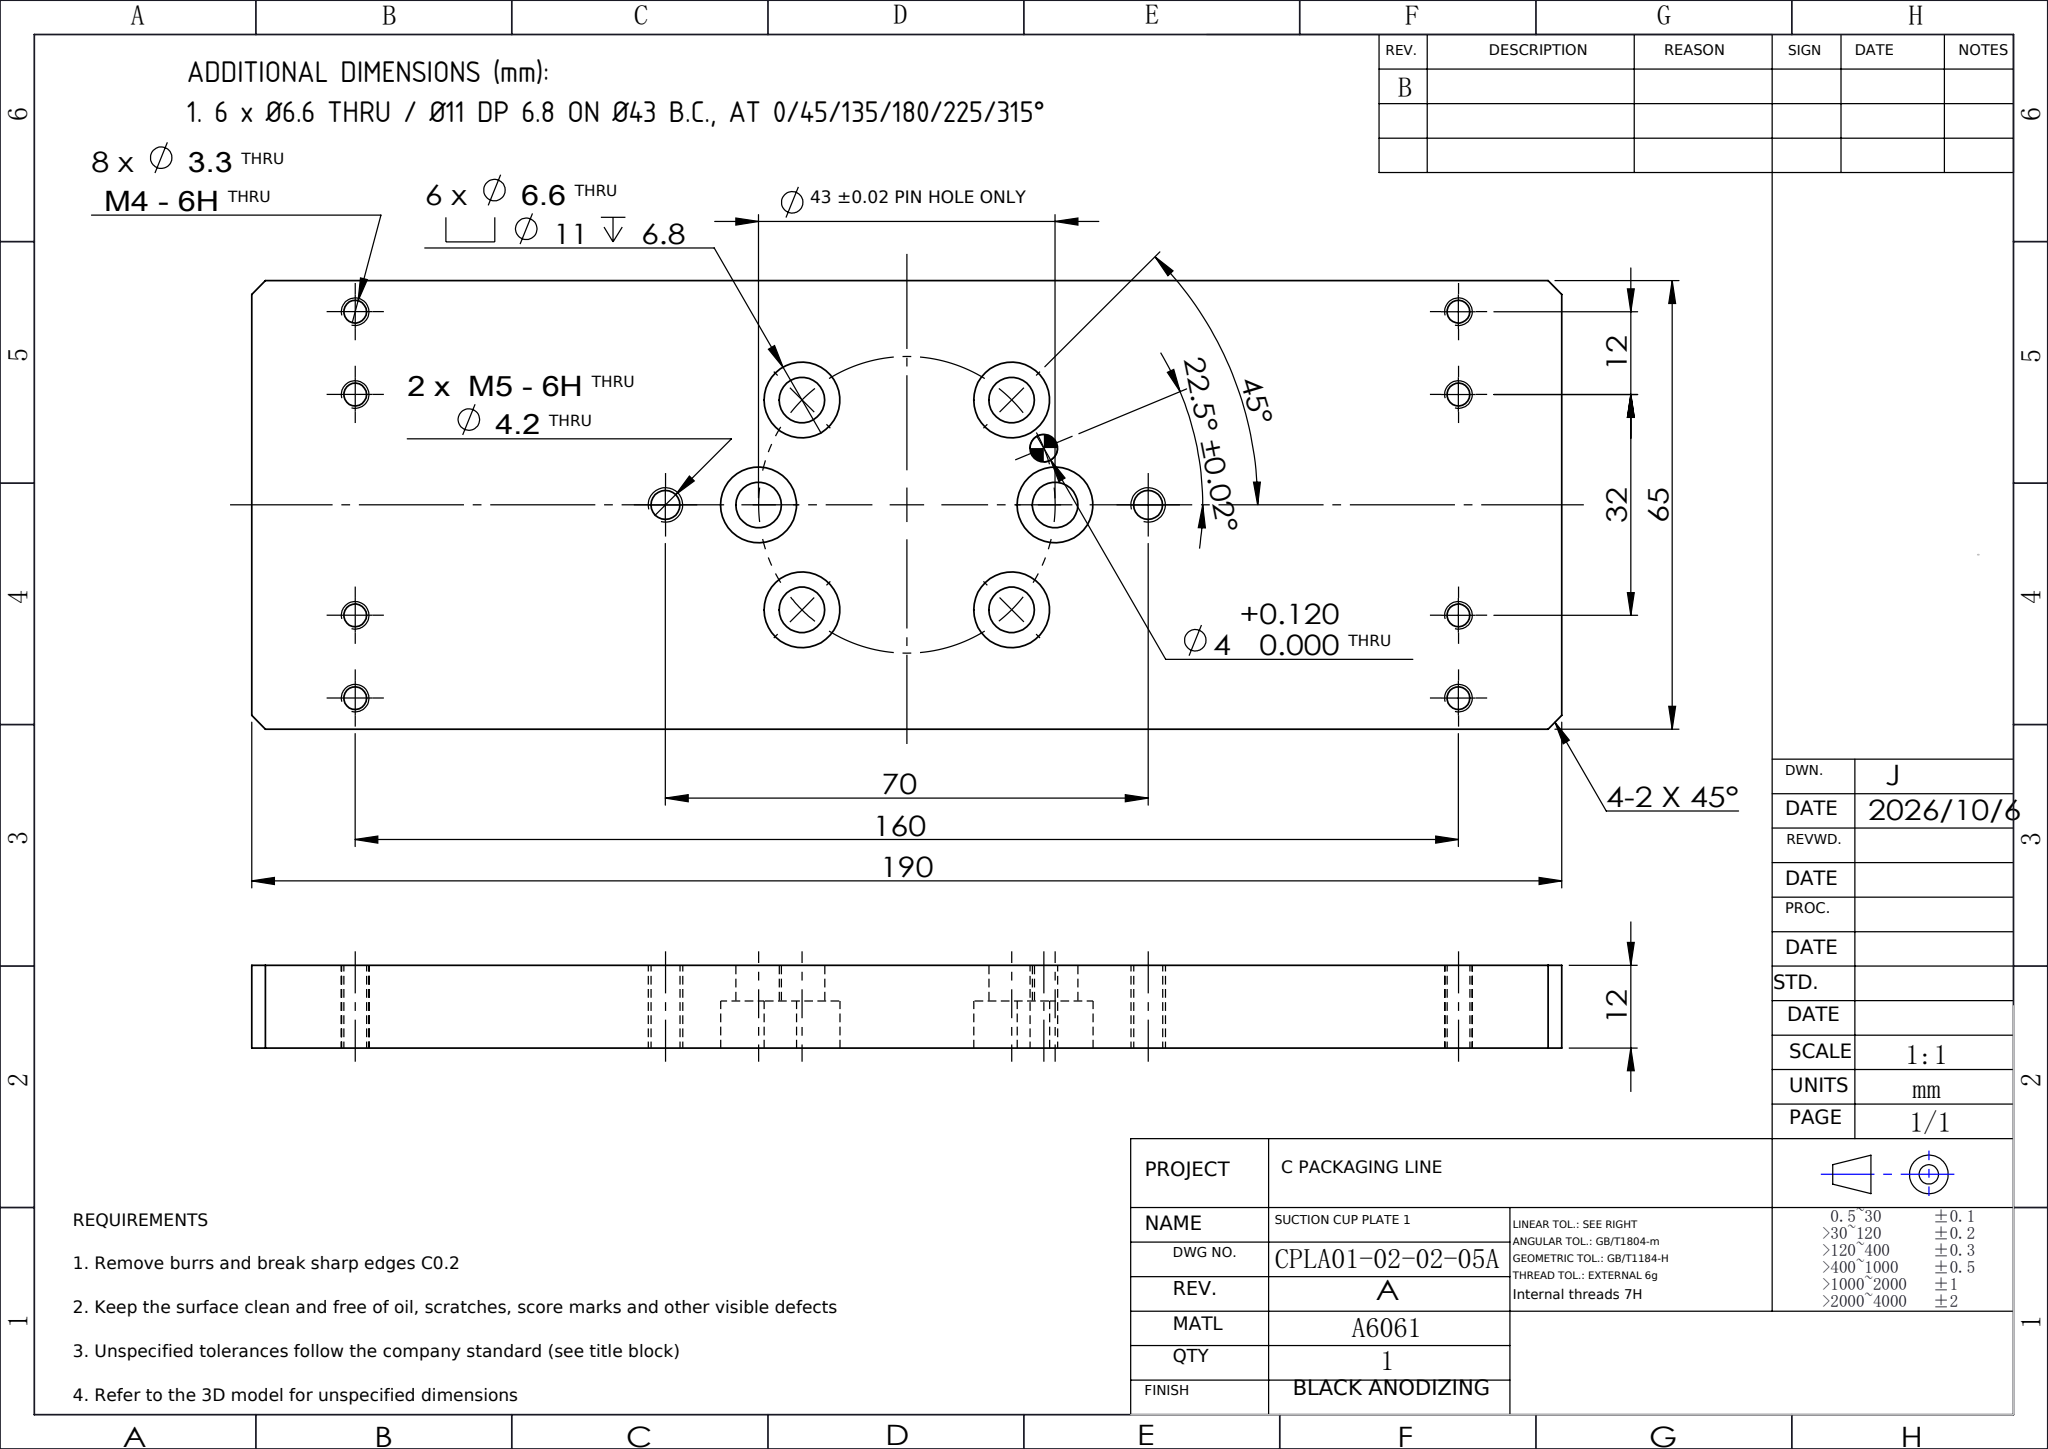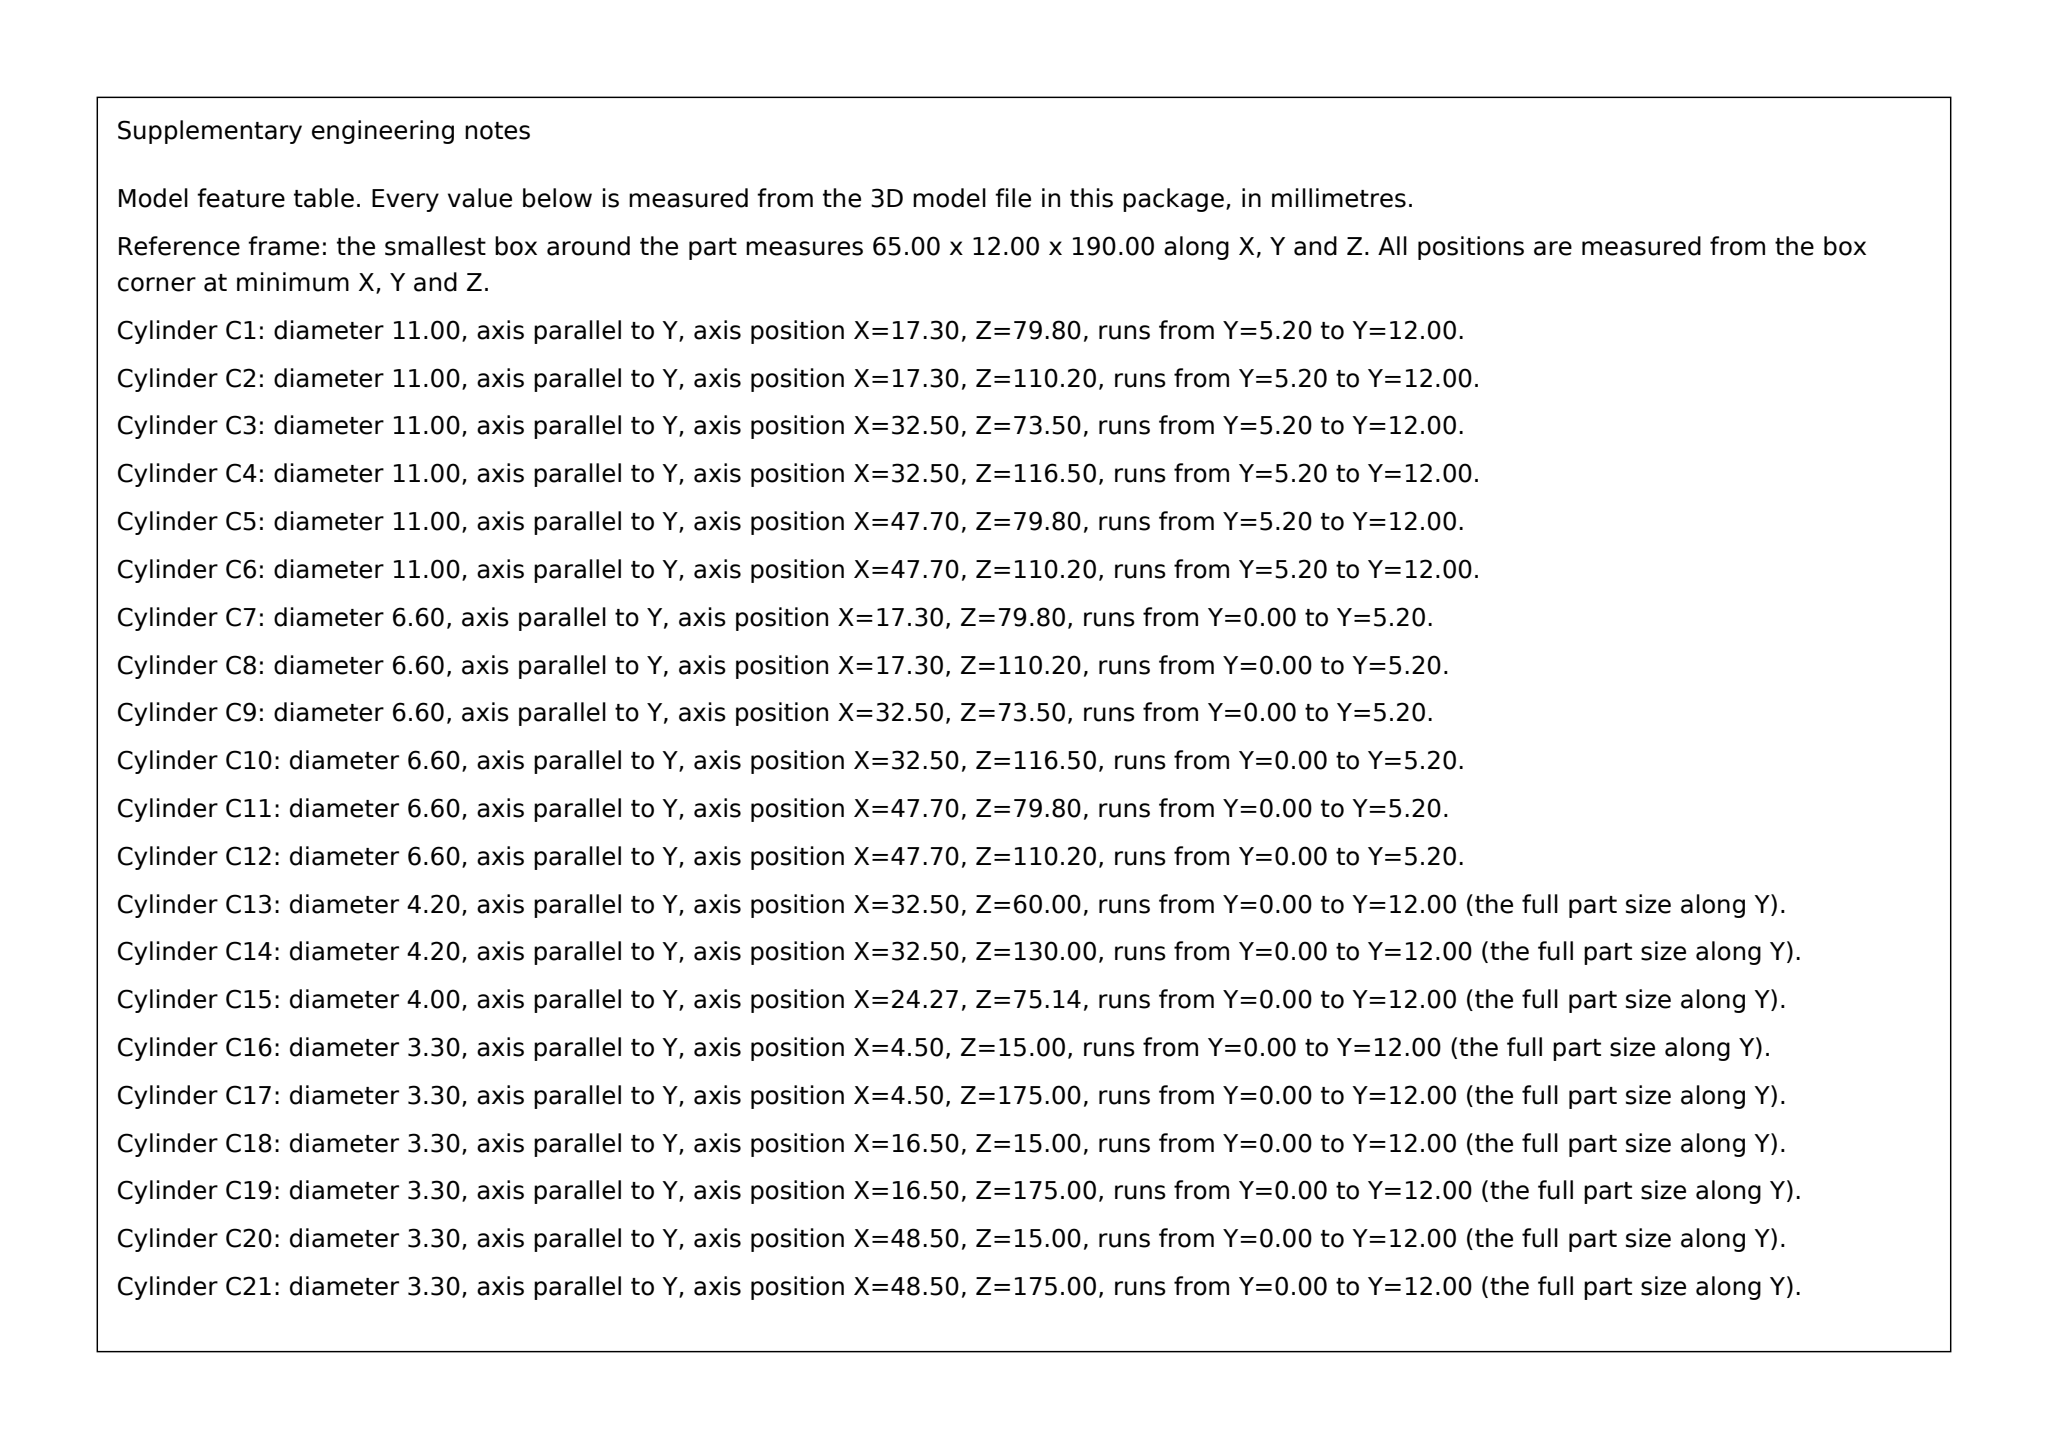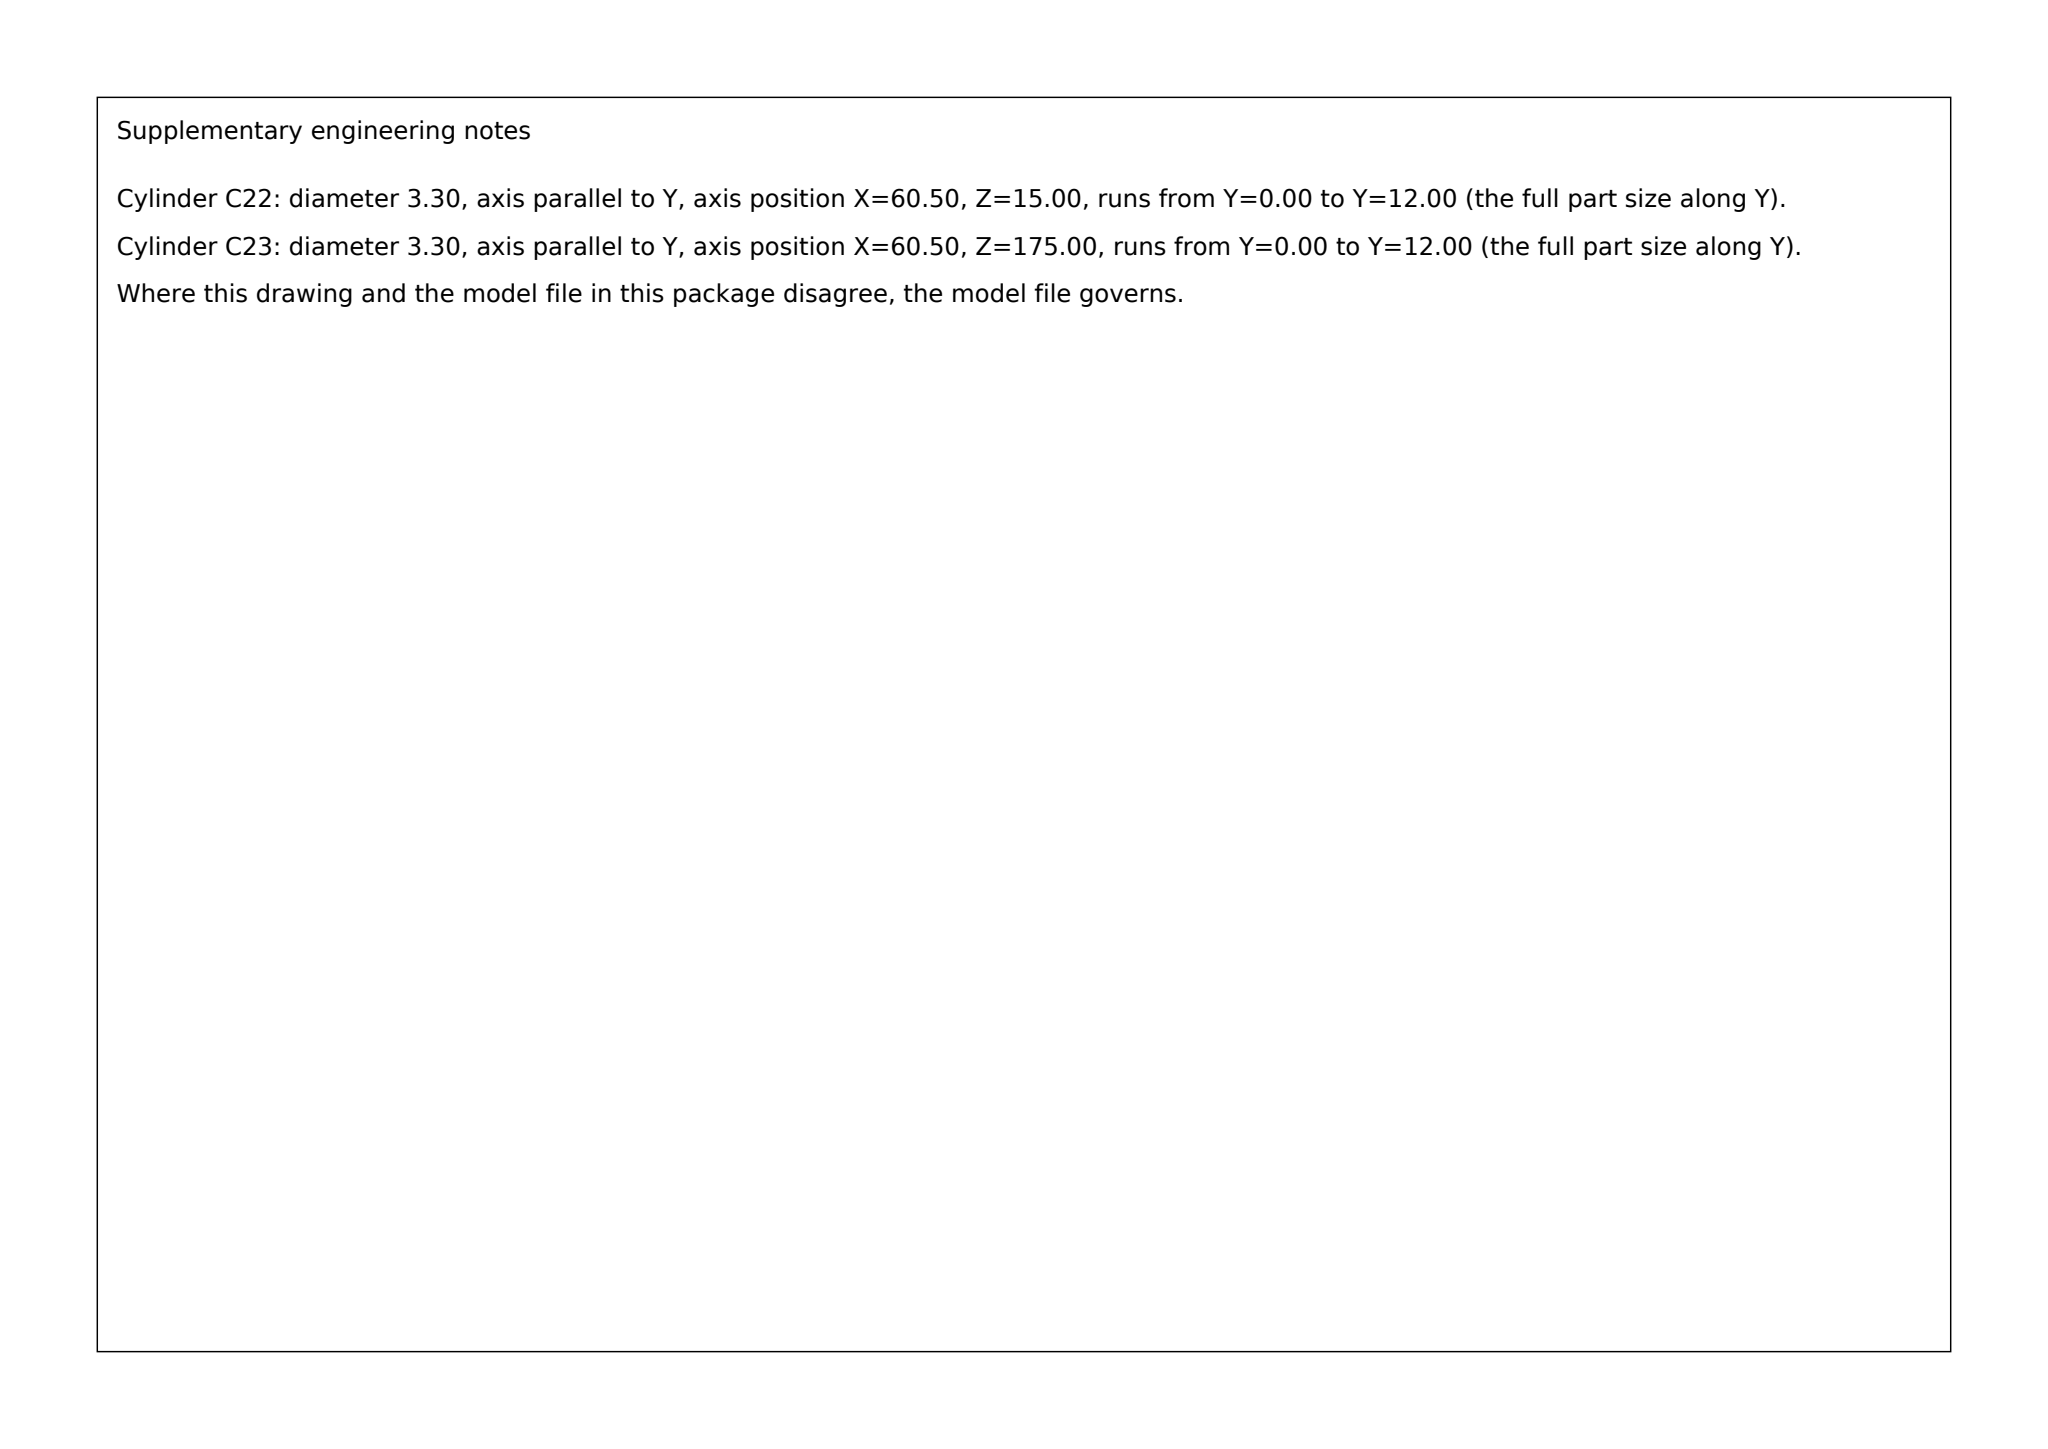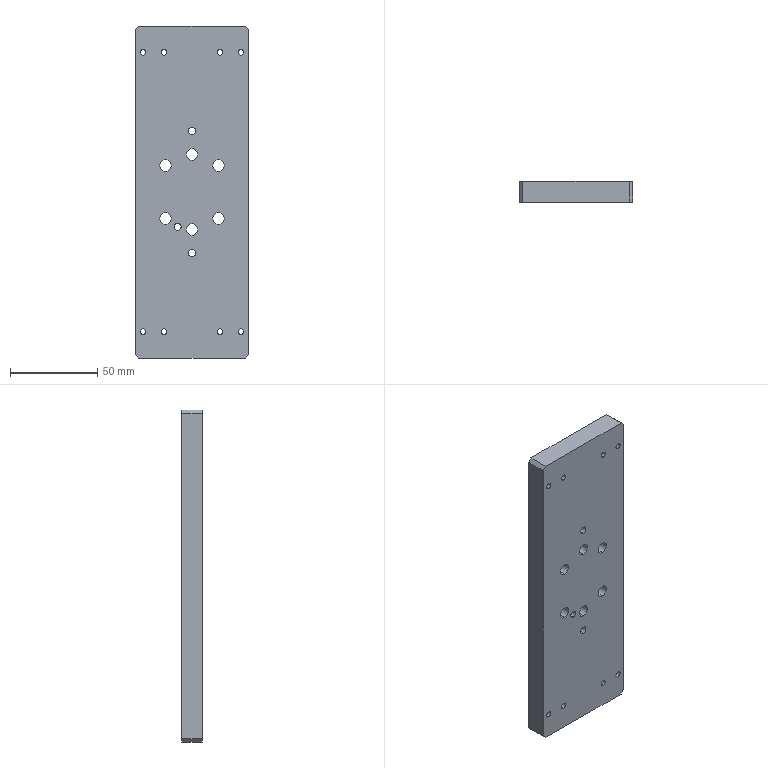Part | SolidWorks | mm | 1 solid | 62 faces | box 65 x 12 x 190 mm | volume 141855 mm3 | cylinder 46 | plane 16 | commonest cylinder face diameters 3.3 x16 11 x12 6.6 x12 4.2 x4 4 x2
build123d program:
from build123d import *

# Parameters (mm, degrees)
SKETCH1_W                                       = 120
SKETCH1_H                                       = 295
BOSS_EXTRUDE1_DEPTH                             = 12
SKETCH2_W                                       = 280
SKETCH2_H                                       = 12
BOSS_EXTRUDE2_DEPTH                             = 55
SKETCH3_R                                       = 6.5
CUT_EXTRUDE1_DEPTH                              = 188.417
LPATTERN1_COUNT                                 = 4
LPATTERN1_PITCH                                 = 68
SKETCH4_W                                       = 12
SKETCH4_H                                       = 2
CUT_EXTRUDE2_DEPTH                              = 230.184
M5_HEX_SOCKET_HEAD_CAP_SCREW_CBORE2_D           = 5.5
M5_HEX_SOCKET_HEAD_CAP_SCREW_CBORE2_CBORE_D     = 10
M5_HEX_SOCKET_HEAD_CAP_SCREW_CBORE2_CBORE_DEPTH = 5.4
SKETCH15_W                                      = 140
SKETCH15_H                                      = 354.743
SKETCH15_W_2                                    = 206.533
SKETCH15_H_2                                    = 375.74
CUT_EXTRUDE3_DEPTH                              = 188.417
SKETCH16_W                                      = 25
SKETCH16_H                                      = 520
CUT_EXTRUDE4_DEPTH                              = 155.678
CHAMFER1_SIZE                                   = 2
FILLET1_R                                       = 5
M4_TAPPED_HOLE1_D                               = 3.3
LPATTERN2_COUNT                                 = 2
LPATTERN2_PITCH                                 = 160
M4_TAPPED_HOLE2_D                               = 3.3
F_5_0MM_DOWEL_PIN_HOLE1_D                       = 5
SKETCH28_W                                      = 171.475
SKETCH28_H                                      = 89.112
CUT_EXTRUDE5_DEPTH                              = 155.678
CHAMFER2_SIZE                                   = 2
SKETCH29_W                                      = 120.267
SKETCH29_H                                      = 29.757
SKETCH29_W_2                                    = 113.82
SKETCH29_H_2                                    = 23.557
CUT_EXTRUDE6_DEPTH                              = 152.514
CHAMFER3_SIZE                                   = 2
SKETCH30_W                                      = 37.387
SKETCH30_H                                      = 12.641
SKETCH30_W_2                                    = 6.59
SKETCH30_H_2                                    = 8.943
SKETCH30_W_3                                    = 6.724
SKETCH30_H_3                                    = 9.279
BOSS_EXTRUDE3_DEPTH                             = 12
M6_HEX_SOCKET_HEAD_CAP_SCREW_CBORE1_D           = 6.6
M6_HEX_SOCKET_HEAD_CAP_SCREW_CBORE1_CBORE_D     = 11
M6_HEX_SOCKET_HEAD_CAP_SCREW_CBORE1_CBORE_DEPTH = 6.8
SKETCH33_R                                      = 2
CUT_EXTRUDE7_DEPTH                              = 133.123
M5_TAPPED_HOLE1_D                               = 4.2


with BuildPart() as part:
    # Sketch1 → Boss-Extrude1 (new body)
    with BuildSketch(Plane(origin=(0, 0, 0), x_dir=(1, 0, 0), z_dir=(0, 1, 0))):
        Rectangle(SKETCH1_W, SKETCH1_H)
    extrude(amount=BOSS_EXTRUDE1_DEPTH)

    # Sketch2 → Boss-Extrude2 (add)
    with BuildSketch(Plane(origin=(60, 0, 0), x_dir=(0, 0, -1), z_dir=(1, 0, 0))):
        with Locations((-7.5, 6)):
            Rectangle(SKETCH2_W, SKETCH2_H)
    boss_extrude2 = extrude(amount=BOSS_EXTRUDE2_DEPTH)

    # Mirror1: Boss-Extrude2 across plane
    add(boss_extrude2.mirror(Plane(origin=(0, 0, 0), x_dir=(0, 0, 1), z_dir=(1, 0, 0))))

    # Sketch3 → Cut-Extrude1 (cut, symmetric)
    with BuildSketch(Plane.XZ):
        with Locations(Location((-60, -79, 0), (0, 0, 270))):
            Circle(SKETCH3_R)
        with Locations(Location((60, -79, 0), (0, 0, 270))):
            Circle(SKETCH3_R)
    cut_extrude1 = extrude(amount=CUT_EXTRUDE1_DEPTH, both=True, mode=Mode.SUBTRACT)

    # LPattern1: Cut-Extrude1 ×4
    with Locations(*[(0, 0, i * LPATTERN1_PITCH) for i in range(1, LPATTERN1_COUNT)]):
        add(cut_extrude1, mode=Mode.SUBTRACT)

    # Sketch4 → Cut-Extrude2 (cut, through all)
    with BuildSketch(Plane.ZY.offset(60)):
        with Locations((-141.5, 1)):
            Rectangle(SKETCH4_W, SKETCH4_H)
    extrude(amount=-CUT_EXTRUDE2_DEPTH, mode=Mode.SUBTRACT)

    # M5 Hex Socket Head Cap Screw CBORE2 (through all)
    with Locations(Plane(origin=(0, 12, 0), x_dir=(1, 0, 0), z_dir=(0, 1, 0))):
        with Locations((0, 141.5), (-37.5, 141.5), (37.5, 141.5)):
            CounterBoreHole(M5_HEX_SOCKET_HEAD_CAP_SCREW_CBORE2_D / 2, M5_HEX_SOCKET_HEAD_CAP_SCREW_CBORE2_CBORE_D / 2, M5_HEX_SOCKET_HEAD_CAP_SCREW_CBORE2_CBORE_DEPTH)

    # Sketch15 → Cut-Extrude3 (cut, through all)
    with BuildSketch(Plane.XZ):
        with Locations((-115, 11.183)):
            Rectangle(SKETCH15_W, SKETCH15_H)
        with Locations((148.267, 21.681)):
            Rectangle(SKETCH15_W_2, SKETCH15_H_2)
    extrude(amount=-CUT_EXTRUDE3_DEPTH, mode=Mode.SUBTRACT)

    # Sketch16 → Cut-Extrude4 (cut, through all)
    with BuildSketch(Plane.XZ):
        with Locations((-45, 147.5)):
            Rectangle(SKETCH16_W, SKETCH16_H)
        with Locations((45, 147.5)):
            Rectangle(SKETCH16_W, SKETCH16_H)
    extrude(amount=-CUT_EXTRUDE4_DEPTH, mode=Mode.SUBTRACT)

    # Chamfer1
    chamfer1_edges = [part.edges().sort_by_distance(p)[0] for p in [
        (-45, 7, -147.5),
        (45, 7, -147.5),
        (-45, 6, -112.5),
        (45, 6, -112.5),
        (-32.5, 6, 147.5),
        (32.5, 6, 147.5),
    ]]
    chamfer(chamfer1_edges, length=CHAMFER1_SIZE)

    # Fillet1
    fillet1_edges = [part.edges().sort_by_distance(p)[0] for p in [
        (-32.5, 6, -112.5),
        (32.5, 6, -112.5),
    ]]
    fillet(fillet1_edges, radius=FILLET1_R)

    # M4 Tapped Hole1 (through all)
    with Locations(Plane(origin=(0, 0, 0), x_dir=(-1, 0, 0), z_dir=(0, -1, 0))):
        with Locations((-28, -112.5), (-16, -112.5), (16, -112.5), (28, -112.5)):
            m4_tapped_hole1 = Hole(M4_TAPPED_HOLE1_D / 2)

    # LPattern2: M4 Tapped Hole1 ×2
    with Locations(*[(0, 0, -i * LPATTERN2_PITCH) for i in range(1, LPATTERN2_COUNT)]):
        add(m4_tapped_hole1, mode=Mode.SUBTRACT)

    # M4 Tapped Hole2 (through all)
    with Locations(Plane(origin=(0, 0, 0), x_dir=(-1, 0, 0), z_dir=(0, -1, 0))):
        with Locations((28, -32.5), (-28, -32.5), (-16, -32.5), (16, -32.5)):
            Hole(M4_TAPPED_HOLE2_D / 2)

    # 5.0mm Dowel Pin Hole1 (through all)
    with Locations(Plane(origin=(0, 12, 0), x_dir=(1, 0, 0), z_dir=(0, 1, 0))):
        with Locations((-18.75, 141.5), (18.75, 141.5)):
            Hole(F_5_0MM_DOWEL_PIN_HOLE1_D / 2)

    # Sketch28 → Cut-Extrude5 (cut, through all)
    with BuildSketch(Plane.XZ):
        with Locations((-0.7914, -127.056)):
            Rectangle(SKETCH28_W, SKETCH28_H)
    extrude(amount=-CUT_EXTRUDE5_DEPTH, mode=Mode.SUBTRACT)

    # Chamfer2
    chamfer2_edges = [part.edges().sort_by_distance(p)[0] for p in [
        (32.5, 6, -82.5),
        (-32.5, 6, -82.5),
    ]]
    chamfer(chamfer2_edges, length=CHAMFER2_SIZE)

    # Sketch29 → Cut-Extrude6 (cut, through all)
    with BuildSketch(Plane.XZ):
        with Locations((3.1, 142.378)):
            Rectangle(SKETCH29_W, SKETCH29_H)
        with Locations((6.323, -74.279)):
            Rectangle(SKETCH29_W_2, SKETCH29_H_2)
    extrude(amount=-CUT_EXTRUDE6_DEPTH, mode=Mode.SUBTRACT)

    # Chamfer3
    chamfer3_edges = [part.edges().sort_by_distance(p)[0] for p in [
        (32.5, 6, -62.5),
        (32.5, 6, 127.5),
        (-32.5, 6, 127.5),
        (-32.5, 6, -62.5),
    ]]
    chamfer(chamfer3_edges, length=CHAMFER3_SIZE)

    # Sketch30 → Boss-Extrude3 (add, through all)
    with BuildSketch(Plane.XZ):
        with Locations((0.03159, 31.271)):
            Rectangle(SKETCH30_W, SKETCH30_H)
        with Locations((27.534, 32.313)):
            Rectangle(SKETCH30_W_2, SKETCH30_H_2)
        with Locations((-28.076, 31.472)):
            Rectangle(SKETCH30_W_3, SKETCH30_H_3)
    extrude(amount=-BOSS_EXTRUDE3_DEPTH)

    # M6 Hex Socket Head Cap Screw CBORE1 (through all)
    with Locations(Plane(origin=(0, 12, 0), x_dir=(1, 0, 0), z_dir=(0, 1, 0))):
        with Locations((15.203, -17.297), (-15.203, -17.297), (0, -11), (15.203, -47.703), (0, -54), (-15.203, -47.703)):
            CounterBoreHole(M6_HEX_SOCKET_HEAD_CAP_SCREW_CBORE1_D / 2, M6_HEX_SOCKET_HEAD_CAP_SCREW_CBORE1_CBORE_D / 2, M6_HEX_SOCKET_HEAD_CAP_SCREW_CBORE1_CBORE_DEPTH)

    # Sketch33 → Cut-Extrude7 (cut, through all)
    with BuildSketch(Plane(origin=(0, 12, 0), x_dir=(1, 0, 0), z_dir=(0, 1, 0))):
        with Locations(Location((-8.228, -12.637, 0), (0, 0, 270))):
            Circle(SKETCH33_R)
    extrude(amount=-CUT_EXTRUDE7_DEPTH, mode=Mode.SUBTRACT)

    # M5 Tapped Hole1 (through all)
    with Locations(Plane(origin=(0, 12, 0), x_dir=(1, 0, 0), z_dir=(0, 1, 0))):
        with Locations((0.000003761, -67.5), (0.000003761, 2.5)):
            Hole(M5_TAPPED_HOLE1_D / 2)


solid = part.part